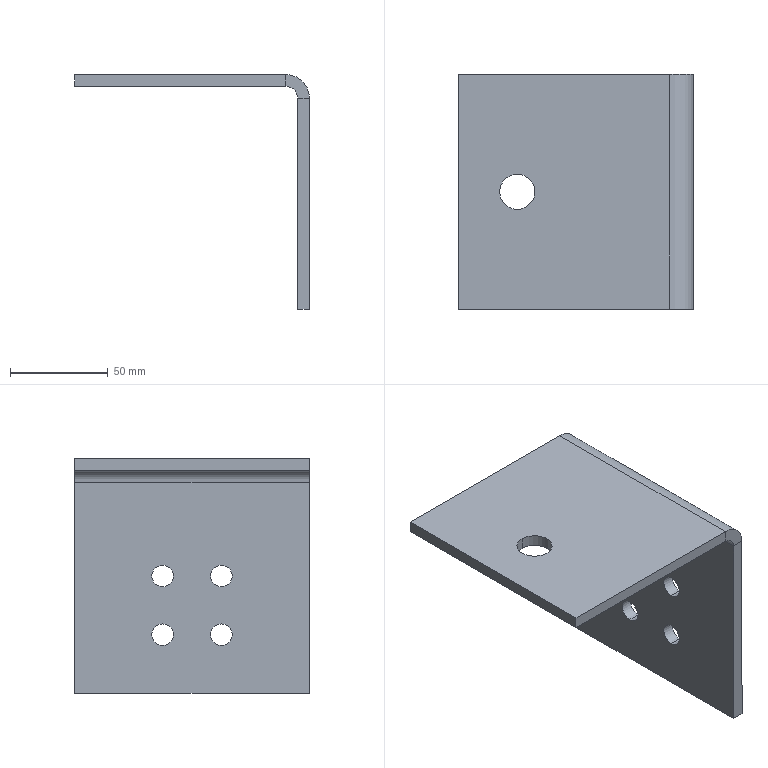Component | SolidWorks | LiftingBentPlate-1 | 1 solid | 24 faces | box 120 x 120 x 120 mm | volume 161891 mm3 | cylinder 12 | plane 12 | commonest cylinder face diameters 11 x8 18 x2 24 x1 12 x1
STEP:
#1=COLOUR_RGB('',0.7922,0.8196,0.9333);
#2=FILL_AREA_STYLE_COLOUR('',#1);
#3=FILL_AREA_STYLE('',(#2));
#4=SURFACE_STYLE_FILL_AREA(#3);
#5=SURFACE_SIDE_STYLE('',(#4));
#6=SURFACE_STYLE_USAGE(.BOTH.,#5);
#7=PRESENTATION_STYLE_ASSIGNMENT((#6));
#8=CARTESIAN_POINT('',(-28.327,8.439,39.587));
#9=VERTEX_POINT('',#8);
#10=CARTESIAN_POINT('',(-28.327,8.439,39.154));
#11=VERTEX_POINT('',#10);
#12=CARTESIAN_POINT('',(-28.327,8.439,39.37));
#13=DIRECTION('',(-1.,0.,0.));
#14=DIRECTION('',(0.,0.,1.));
#15=AXIS2_PLACEMENT_3D('',#12,#13,#14);
#16=CIRCLE('',#15,0.2165);
#17=EDGE_CURVE('',#9,#11,#16,.T.);
#18=ORIENTED_EDGE('',*,*,#17,.T.);
#19=CARTESIAN_POINT('',(-28.091,8.439,39.154));
#20=VERTEX_POINT('',#19);
#21=CARTESIAN_POINT('',(-32.815,8.439,39.154));
#22=DIRECTION('',(1.,-0.,-0.));
#23=VECTOR('',#22,39.37);
#24=LINE('',#21,#23);
#25=EDGE_CURVE('',#11,#20,#24,.T.);
#26=ORIENTED_EDGE('',*,*,#25,.T.);
#27=CARTESIAN_POINT('',(-28.091,8.439,39.587));
#28=VERTEX_POINT('',#27);
#29=CARTESIAN_POINT('',(-28.091,8.439,39.37));
#30=DIRECTION('',(1.,-0.,-0.));
#31=DIRECTION('',(0.,0.,1.));
#32=AXIS2_PLACEMENT_3D('',#29,#30,#31);
#33=CIRCLE('',#32,0.2165);
#34=EDGE_CURVE('',#20,#28,#33,.T.);
#35=ORIENTED_EDGE('',*,*,#34,.T.);
#36=CARTESIAN_POINT('',(-32.815,8.439,39.587));
#37=DIRECTION('',(1.,-0.,-0.));
#38=VECTOR('',#37,39.37);
#39=LINE('',#36,#38);
#40=EDGE_CURVE('',#9,#28,#39,.T.);
#41=ORIENTED_EDGE('',*,*,#40,.F.);
#42=EDGE_LOOP('',(#18,#26,#35,#41));
#43=FACE_OUTER_BOUND('',#42,.T.);
#44=CARTESIAN_POINT('',(-32.815,8.439,39.37));
#45=DIRECTION('',(1.,-0.,-0.));
#46=DIRECTION('',(0.,0.,1.));
#47=AXIS2_PLACEMENT_3D('',#44,#45,#46);
#48=CYLINDRICAL_SURFACE('',#47,0.2165);
#49=ADVANCED_FACE('',(#43),#48,.F.);
#50=CARTESIAN_POINT('',(-28.327,7.258,39.587));
#51=VERTEX_POINT('',#50);
#52=CARTESIAN_POINT('',(-28.327,7.258,39.154));
#53=VERTEX_POINT('',#52);
#54=CARTESIAN_POINT('',(-28.327,7.258,39.37));
#55=DIRECTION('',(-1.,0.,0.));
#56=DIRECTION('',(0.,0.,1.));
#57=AXIS2_PLACEMENT_3D('',#54,#55,#56);
#58=CIRCLE('',#57,0.2165);
#59=EDGE_CURVE('',#51,#53,#58,.T.);
#60=ORIENTED_EDGE('',*,*,#59,.T.);
#61=CARTESIAN_POINT('',(-28.091,7.258,39.154));
#62=VERTEX_POINT('',#61);
#63=CARTESIAN_POINT('',(-32.815,7.258,39.154));
#64=DIRECTION('',(1.,-0.,-0.));
#65=VECTOR('',#64,39.37);
#66=LINE('',#63,#65);
#67=EDGE_CURVE('',#53,#62,#66,.T.);
#68=ORIENTED_EDGE('',*,*,#67,.T.);
#69=CARTESIAN_POINT('',(-28.091,7.258,39.587));
#70=VERTEX_POINT('',#69);
#71=CARTESIAN_POINT('',(-28.091,7.258,39.37));
#72=DIRECTION('',(1.,-0.,-0.));
#73=DIRECTION('',(0.,0.,1.));
#74=AXIS2_PLACEMENT_3D('',#71,#72,#73);
#75=CIRCLE('',#74,0.2165);
#76=EDGE_CURVE('',#62,#70,#75,.T.);
#77=ORIENTED_EDGE('',*,*,#76,.T.);
#78=CARTESIAN_POINT('',(-32.815,7.258,39.587));
#79=DIRECTION('',(1.,-0.,-0.));
#80=VECTOR('',#79,39.37);
#81=LINE('',#78,#80);
#82=EDGE_CURVE('',#51,#70,#81,.T.);
#83=ORIENTED_EDGE('',*,*,#82,.F.);
#84=EDGE_LOOP('',(#60,#68,#77,#83));
#85=FACE_OUTER_BOUND('',#84,.T.);
#86=CARTESIAN_POINT('',(-32.815,7.258,39.37));
#87=DIRECTION('',(1.,-0.,-0.));
#88=DIRECTION('',(0.,0.,1.));
#89=AXIS2_PLACEMENT_3D('',#86,#87,#88);
#90=CYLINDRICAL_SURFACE('',#89,0.2165);
#91=ADVANCED_FACE('',(#85),#90,.F.);
#92=CARTESIAN_POINT('',(-28.327,8.439,40.768));
#93=VERTEX_POINT('',#92);
#94=CARTESIAN_POINT('',(-28.327,8.439,40.335));
#95=VERTEX_POINT('',#94);
#96=CARTESIAN_POINT('',(-28.327,8.439,40.551));
#97=DIRECTION('',(-1.,0.,0.));
#98=DIRECTION('',(0.,0.,1.));
#99=AXIS2_PLACEMENT_3D('',#96,#97,#98);
#100=CIRCLE('',#99,0.2165);
#101=EDGE_CURVE('',#93,#95,#100,.T.);
#102=ORIENTED_EDGE('',*,*,#101,.T.);
#103=CARTESIAN_POINT('',(-28.091,8.439,40.335));
#104=VERTEX_POINT('',#103);
#105=CARTESIAN_POINT('',(-32.815,8.439,40.335));
#106=DIRECTION('',(1.,-0.,-0.));
#107=VECTOR('',#106,39.37);
#108=LINE('',#105,#107);
#109=EDGE_CURVE('',#95,#104,#108,.T.);
#110=ORIENTED_EDGE('',*,*,#109,.T.);
#111=CARTESIAN_POINT('',(-28.091,8.439,40.768));
#112=VERTEX_POINT('',#111);
#113=CARTESIAN_POINT('',(-28.091,8.439,40.551));
#114=DIRECTION('',(1.,-0.,-0.));
#115=DIRECTION('',(0.,0.,1.));
#116=AXIS2_PLACEMENT_3D('',#113,#114,#115);
#117=CIRCLE('',#116,0.2165);
#118=EDGE_CURVE('',#104,#112,#117,.T.);
#119=ORIENTED_EDGE('',*,*,#118,.T.);
#120=CARTESIAN_POINT('',(-32.815,8.439,40.768));
#121=DIRECTION('',(1.,-0.,-0.));
#122=VECTOR('',#121,39.37);
#123=LINE('',#120,#122);
#124=EDGE_CURVE('',#93,#112,#123,.T.);
#125=ORIENTED_EDGE('',*,*,#124,.F.);
#126=EDGE_LOOP('',(#102,#110,#119,#125));
#127=FACE_OUTER_BOUND('',#126,.T.);
#128=CARTESIAN_POINT('',(-32.815,8.439,40.551));
#129=DIRECTION('',(1.,-0.,-0.));
#130=DIRECTION('',(0.,0.,1.));
#131=AXIS2_PLACEMENT_3D('',#128,#129,#130);
#132=CYLINDRICAL_SURFACE('',#131,0.2165);
#133=ADVANCED_FACE('',(#127),#132,.F.);
#134=CARTESIAN_POINT('',(-28.327,7.258,40.768));
#135=VERTEX_POINT('',#134);
#136=CARTESIAN_POINT('',(-28.327,7.258,40.335));
#137=VERTEX_POINT('',#136);
#138=CARTESIAN_POINT('',(-28.327,7.258,40.551));
#139=DIRECTION('',(-1.,0.,0.));
#140=DIRECTION('',(0.,0.,1.));
#141=AXIS2_PLACEMENT_3D('',#138,#139,#140);
#142=CIRCLE('',#141,0.2165);
#143=EDGE_CURVE('',#135,#137,#142,.T.);
#144=ORIENTED_EDGE('',*,*,#143,.T.);
#145=CARTESIAN_POINT('',(-28.091,7.258,40.335));
#146=VERTEX_POINT('',#145);
#147=CARTESIAN_POINT('',(-32.815,7.258,40.335));
#148=DIRECTION('',(1.,-0.,-0.));
#149=VECTOR('',#148,39.37);
#150=LINE('',#147,#149);
#151=EDGE_CURVE('',#137,#146,#150,.T.);
#152=ORIENTED_EDGE('',*,*,#151,.T.);
#153=CARTESIAN_POINT('',(-28.091,7.258,40.768));
#154=VERTEX_POINT('',#153);
#155=CARTESIAN_POINT('',(-28.091,7.258,40.551));
#156=DIRECTION('',(1.,-0.,-0.));
#157=DIRECTION('',(0.,0.,1.));
#158=AXIS2_PLACEMENT_3D('',#155,#156,#157);
#159=CIRCLE('',#158,0.2165);
#160=EDGE_CURVE('',#146,#154,#159,.T.);
#161=ORIENTED_EDGE('',*,*,#160,.T.);
#162=CARTESIAN_POINT('',(-32.815,7.258,40.768));
#163=DIRECTION('',(1.,-0.,-0.));
#164=VECTOR('',#163,39.37);
#165=LINE('',#162,#164);
#166=EDGE_CURVE('',#135,#154,#165,.T.);
#167=ORIENTED_EDGE('',*,*,#166,.F.);
#168=EDGE_LOOP('',(#144,#152,#161,#167));
#169=FACE_OUTER_BOUND('',#168,.T.);
#170=CARTESIAN_POINT('',(-32.815,7.258,40.551));
#171=DIRECTION('',(1.,-0.,-0.));
#172=DIRECTION('',(0.,0.,1.));
#173=AXIS2_PLACEMENT_3D('',#170,#171,#172);
#174=CYLINDRICAL_SURFACE('',#173,0.2165);
#175=ADVANCED_FACE('',(#169),#174,.F.);
#176=CARTESIAN_POINT('',(-31.634,7.494,42.677));
#177=VERTEX_POINT('',#176);
#178=CARTESIAN_POINT('',(-31.634,8.203,42.677));
#179=VERTEX_POINT('',#178);
#180=CARTESIAN_POINT('',(-31.634,7.849,42.677));
#181=DIRECTION('',(-0.,-0.,-1.));
#182=DIRECTION('',(-0.,-1.,0.));
#183=AXIS2_PLACEMENT_3D('',#180,#181,#182);
#184=CIRCLE('',#183,0.3543);
#185=EDGE_CURVE('',#177,#179,#184,.T.);
#186=ORIENTED_EDGE('',*,*,#185,.T.);
#187=CARTESIAN_POINT('',(-31.634,8.203,42.913));
#188=VERTEX_POINT('',#187);
#189=CARTESIAN_POINT('',(-31.634,8.203,38.189));
#190=DIRECTION('',(0.,0.,1.));
#191=VECTOR('',#190,39.37);
#192=LINE('',#189,#191);
#193=EDGE_CURVE('',#179,#188,#192,.T.);
#194=ORIENTED_EDGE('',*,*,#193,.T.);
#195=CARTESIAN_POINT('',(-31.634,7.494,42.913));
#196=VERTEX_POINT('',#195);
#197=CARTESIAN_POINT('',(-31.634,7.849,42.913));
#198=DIRECTION('',(0.,0.,1.));
#199=DIRECTION('',(-0.,-1.,0.));
#200=AXIS2_PLACEMENT_3D('',#197,#198,#199);
#201=CIRCLE('',#200,0.3543);
#202=EDGE_CURVE('',#188,#196,#201,.T.);
#203=ORIENTED_EDGE('',*,*,#202,.T.);
#204=CARTESIAN_POINT('',(-31.634,7.494,38.189));
#205=DIRECTION('',(0.,0.,1.));
#206=VECTOR('',#205,39.37);
#207=LINE('',#204,#206);
#208=EDGE_CURVE('',#177,#196,#207,.T.);
#209=ORIENTED_EDGE('',*,*,#208,.F.);
#210=EDGE_LOOP('',(#186,#194,#203,#209));
#211=FACE_OUTER_BOUND('',#210,.T.);
#212=CARTESIAN_POINT('',(-31.634,7.849,38.189));
#213=DIRECTION('',(0.,0.,1.));
#214=DIRECTION('',(-0.,-1.,0.));
#215=AXIS2_PLACEMENT_3D('',#212,#213,#214);
#216=CYLINDRICAL_SURFACE('',#215,0.3543);
#217=ADVANCED_FACE('',(#211),#216,.F.);
#218=CARTESIAN_POINT('',(-28.091,5.486,42.441));
#219=VERTEX_POINT('',#218);
#220=CARTESIAN_POINT('',(-28.327,5.486,42.441));
#221=VERTEX_POINT('',#220);
#222=CARTESIAN_POINT('',(-28.091,5.486,42.441));
#223=DIRECTION('',(-1.,0.,0.));
#224=VECTOR('',#223,39.37);
#225=LINE('',#222,#224);
#226=EDGE_CURVE('',#219,#221,#225,.T.);
#227=ORIENTED_EDGE('',*,*,#226,.F.);
#228=CARTESIAN_POINT('',(-28.563,5.486,42.913));
#229=VERTEX_POINT('',#228);
#230=CARTESIAN_POINT('',(-28.563,5.486,42.441));
#231=DIRECTION('',(0.,1.,-0.));
#232=DIRECTION('',(1.,-0.,0.));
#233=AXIS2_PLACEMENT_3D('',#230,#231,#232);
#234=CIRCLE('',#233,0.4724);
#235=EDGE_CURVE('',#229,#219,#234,.T.);
#236=ORIENTED_EDGE('',*,*,#235,.F.);
#237=CARTESIAN_POINT('',(-28.563,5.486,42.677));
#238=VERTEX_POINT('',#237);
#239=CARTESIAN_POINT('',(-28.563,5.486,42.677));
#240=DIRECTION('',(0.,0.,1.));
#241=VECTOR('',#240,39.37);
#242=LINE('',#239,#241);
#243=EDGE_CURVE('',#238,#229,#242,.T.);
#244=ORIENTED_EDGE('',*,*,#243,.F.);
#245=CARTESIAN_POINT('',(-28.563,5.486,42.441));
#246=DIRECTION('',(0.,1.,-0.));
#247=DIRECTION('',(1.,-0.,0.));
#248=AXIS2_PLACEMENT_3D('',#245,#246,#247);
#249=CIRCLE('',#248,0.2362);
#250=EDGE_CURVE('',#238,#221,#249,.T.);
#251=ORIENTED_EDGE('',*,*,#250,.T.);
#252=EDGE_LOOP('',(#227,#236,#244,#251));
#253=FACE_OUTER_BOUND('',#252,.T.);
#254=CARTESIAN_POINT('',(-28.091,5.486,42.441));
#255=DIRECTION('',(-0.,-1.,0.));
#256=DIRECTION('',(1.,-0.,-0.));
#257=AXIS2_PLACEMENT_3D('',#254,#255,#256);
#258=PLANE('',#257);
#259=ADVANCED_FACE('',(#253),#258,.T.);
#260=CARTESIAN_POINT('',(-28.091,5.486,38.189));
#261=VERTEX_POINT('',#260);
#262=CARTESIAN_POINT('',(-28.091,5.486,42.913));
#263=DIRECTION('',(-0.,-0.,-1.));
#264=VECTOR('',#263,39.37);
#265=LINE('',#262,#264);
#266=EDGE_CURVE('',#219,#261,#265,.T.);
#267=ORIENTED_EDGE('',*,*,#266,.F.);
#268=ORIENTED_EDGE('',*,*,#226,.T.);
#269=CARTESIAN_POINT('',(-28.327,5.486,38.189));
#270=VERTEX_POINT('',#269);
#271=CARTESIAN_POINT('',(-28.327,5.486,42.913));
#272=DIRECTION('',(-0.,-0.,-1.));
#273=VECTOR('',#272,39.37);
#274=LINE('',#271,#273);
#275=EDGE_CURVE('',#221,#270,#274,.T.);
#276=ORIENTED_EDGE('',*,*,#275,.T.);
#277=CARTESIAN_POINT('',(-28.091,5.486,38.189));
#278=DIRECTION('',(-1.,0.,0.));
#279=VECTOR('',#278,39.37);
#280=LINE('',#277,#279);
#281=EDGE_CURVE('',#261,#270,#280,.T.);
#282=ORIENTED_EDGE('',*,*,#281,.F.);
#283=EDGE_LOOP('',(#267,#268,#276,#282));
#284=FACE_OUTER_BOUND('',#283,.T.);
#285=CARTESIAN_POINT('',(-28.563,5.486,42.677));
#286=DIRECTION('',(-0.,-1.,0.));
#287=DIRECTION('',(1.,-0.,-0.));
#288=AXIS2_PLACEMENT_3D('',#285,#286,#287);
#289=PLANE('',#288);
#290=ADVANCED_FACE('',(#284),#289,.T.);
#291=CARTESIAN_POINT('',(-28.563,10.211,42.913));
#292=VERTEX_POINT('',#291);
#293=CARTESIAN_POINT('',(-28.563,10.211,42.677));
#294=VERTEX_POINT('',#293);
#295=CARTESIAN_POINT('',(-28.563,10.211,42.913));
#296=DIRECTION('',(-0.,-0.,-1.));
#297=VECTOR('',#296,39.37);
#298=LINE('',#295,#297);
#299=EDGE_CURVE('',#292,#294,#298,.T.);
#300=ORIENTED_EDGE('',*,*,#299,.F.);
#301=CARTESIAN_POINT('',(-28.091,10.211,42.441));
#302=VERTEX_POINT('',#301);
#303=CARTESIAN_POINT('',(-28.563,10.211,42.441));
#304=DIRECTION('',(0.,1.,-0.));
#305=DIRECTION('',(1.,-0.,0.));
#306=AXIS2_PLACEMENT_3D('',#303,#304,#305);
#307=CIRCLE('',#306,0.4724);
#308=EDGE_CURVE('',#292,#302,#307,.T.);
#309=ORIENTED_EDGE('',*,*,#308,.T.);
#310=CARTESIAN_POINT('',(-28.327,10.211,42.441));
#311=VERTEX_POINT('',#310);
#312=CARTESIAN_POINT('',(-28.327,10.211,42.441));
#313=DIRECTION('',(1.,-0.,-0.));
#314=VECTOR('',#313,39.37);
#315=LINE('',#312,#314);
#316=EDGE_CURVE('',#311,#302,#315,.T.);
#317=ORIENTED_EDGE('',*,*,#316,.F.);
#318=CARTESIAN_POINT('',(-28.563,10.211,42.441));
#319=DIRECTION('',(0.,1.,-0.));
#320=DIRECTION('',(1.,-0.,0.));
#321=AXIS2_PLACEMENT_3D('',#318,#319,#320);
#322=CIRCLE('',#321,0.2362);
#323=EDGE_CURVE('',#294,#311,#322,.T.);
#324=ORIENTED_EDGE('',*,*,#323,.F.);
#325=EDGE_LOOP('',(#300,#309,#317,#324));
#326=FACE_OUTER_BOUND('',#325,.T.);
#327=CARTESIAN_POINT('',(-28.563,10.211,42.913));
#328=DIRECTION('',(0.,1.,-0.));
#329=DIRECTION('',(-1.,0.,0.));
#330=AXIS2_PLACEMENT_3D('',#327,#328,#329);
#331=PLANE('',#330);
#332=ADVANCED_FACE('',(#326),#331,.T.);
#333=CARTESIAN_POINT('',(-32.815,10.211,42.913));
#334=VERTEX_POINT('',#333);
#335=CARTESIAN_POINT('',(-32.815,10.211,42.913));
#336=DIRECTION('',(1.,-0.,-0.));
#337=VECTOR('',#336,39.37);
#338=LINE('',#335,#337);
#339=EDGE_CURVE('',#334,#292,#338,.T.);
#340=ORIENTED_EDGE('',*,*,#339,.T.);
#341=ORIENTED_EDGE('',*,*,#299,.T.);
#342=CARTESIAN_POINT('',(-32.815,10.211,42.677));
#343=VERTEX_POINT('',#342);
#344=CARTESIAN_POINT('',(-32.815,10.211,42.677));
#345=DIRECTION('',(1.,-0.,-0.));
#346=VECTOR('',#345,39.37);
#347=LINE('',#344,#346);
#348=EDGE_CURVE('',#343,#294,#347,.T.);
#349=ORIENTED_EDGE('',*,*,#348,.F.);
#350=CARTESIAN_POINT('',(-32.815,10.211,42.677));
#351=DIRECTION('',(0.,0.,1.));
#352=VECTOR('',#351,39.37);
#353=LINE('',#350,#352);
#354=EDGE_CURVE('',#343,#334,#353,.T.);
#355=ORIENTED_EDGE('',*,*,#354,.T.);
#356=EDGE_LOOP('',(#340,#341,#349,#355));
#357=FACE_OUTER_BOUND('',#356,.T.);
#358=CARTESIAN_POINT('',(-28.327,10.211,42.441));
#359=DIRECTION('',(0.,1.,-0.));
#360=DIRECTION('',(-1.,0.,0.));
#361=AXIS2_PLACEMENT_3D('',#358,#359,#360);
#362=PLANE('',#361);
#363=ADVANCED_FACE('',(#357),#362,.T.);
#364=ORIENTED_EDGE('',*,*,#17,.F.);
#365=CARTESIAN_POINT('',(-28.327,8.439,39.37));
#366=DIRECTION('',(-1.,0.,0.));
#367=DIRECTION('',(0.,0.,1.));
#368=AXIS2_PLACEMENT_3D('',#365,#366,#367);
#369=CIRCLE('',#368,0.2165);
#370=EDGE_CURVE('',#11,#9,#369,.T.);
#371=ORIENTED_EDGE('',*,*,#370,.F.);
#372=EDGE_LOOP('',(#364,#371));
#373=FACE_BOUND('',#372,.T.);
#374=ORIENTED_EDGE('',*,*,#59,.F.);
#375=CARTESIAN_POINT('',(-28.327,7.258,39.37));
#376=DIRECTION('',(-1.,0.,0.));
#377=DIRECTION('',(0.,0.,1.));
#378=AXIS2_PLACEMENT_3D('',#375,#376,#377);
#379=CIRCLE('',#378,0.2165);
#380=EDGE_CURVE('',#53,#51,#379,.T.);
#381=ORIENTED_EDGE('',*,*,#380,.F.);
#382=EDGE_LOOP('',(#374,#381));
#383=FACE_BOUND('',#382,.T.);
#384=ORIENTED_EDGE('',*,*,#101,.F.);
#385=CARTESIAN_POINT('',(-28.327,8.439,40.551));
#386=DIRECTION('',(-1.,0.,0.));
#387=DIRECTION('',(0.,0.,1.));
#388=AXIS2_PLACEMENT_3D('',#385,#386,#387);
#389=CIRCLE('',#388,0.2165);
#390=EDGE_CURVE('',#95,#93,#389,.T.);
#391=ORIENTED_EDGE('',*,*,#390,.F.);
#392=EDGE_LOOP('',(#384,#391));
#393=FACE_BOUND('',#392,.T.);
#394=ORIENTED_EDGE('',*,*,#143,.F.);
#395=CARTESIAN_POINT('',(-28.327,7.258,40.551));
#396=DIRECTION('',(-1.,0.,0.));
#397=DIRECTION('',(0.,0.,1.));
#398=AXIS2_PLACEMENT_3D('',#395,#396,#397);
#399=CIRCLE('',#398,0.2165);
#400=EDGE_CURVE('',#137,#135,#399,.T.);
#401=ORIENTED_EDGE('',*,*,#400,.F.);
#402=EDGE_LOOP('',(#394,#401));
#403=FACE_BOUND('',#402,.T.);
#404=CARTESIAN_POINT('',(-28.327,10.211,38.189));
#405=VERTEX_POINT('',#404);
#406=CARTESIAN_POINT('',(-28.327,10.211,42.913));
#407=DIRECTION('',(-0.,-0.,-1.));
#408=VECTOR('',#407,39.37);
#409=LINE('',#406,#408);
#410=EDGE_CURVE('',#311,#405,#409,.T.);
#411=ORIENTED_EDGE('',*,*,#410,.T.);
#412=CARTESIAN_POINT('',(-28.327,5.486,38.189));
#413=DIRECTION('',(0.,1.,-0.));
#414=VECTOR('',#413,39.37);
#415=LINE('',#412,#414);
#416=EDGE_CURVE('',#270,#405,#415,.T.);
#417=ORIENTED_EDGE('',*,*,#416,.F.);
#418=ORIENTED_EDGE('',*,*,#275,.F.);
#419=CARTESIAN_POINT('',(-28.327,5.486,42.441));
#420=DIRECTION('',(0.,1.,-0.));
#421=VECTOR('',#420,39.37);
#422=LINE('',#419,#421);
#423=EDGE_CURVE('',#221,#311,#422,.T.);
#424=ORIENTED_EDGE('',*,*,#423,.T.);
#425=EDGE_LOOP('',(#411,#417,#418,#424));
#426=FACE_OUTER_BOUND('',#425,.T.);
#427=CARTESIAN_POINT('',(-28.327,5.486,42.913));
#428=DIRECTION('',(1.,-0.,-0.));
#429=DIRECTION('',(0.,0.,1.));
#430=AXIS2_PLACEMENT_3D('',#427,#428,#429);
#431=PLANE('',#430);
#432=ADVANCED_FACE('',(#373,#383,#393,#403,#426),#431,.F.);
#433=CARTESIAN_POINT('',(-28.091,10.211,38.189));
#434=VERTEX_POINT('',#433);
#435=CARTESIAN_POINT('',(-28.091,10.211,38.189));
#436=DIRECTION('',(-1.,0.,0.));
#437=VECTOR('',#436,39.37);
#438=LINE('',#435,#437);
#439=EDGE_CURVE('',#434,#405,#438,.T.);
#440=ORIENTED_EDGE('',*,*,#439,.F.);
#441=CARTESIAN_POINT('',(-28.091,5.486,38.189));
#442=DIRECTION('',(0.,1.,-0.));
#443=VECTOR('',#442,39.37);
#444=LINE('',#441,#443);
#445=EDGE_CURVE('',#261,#434,#444,.T.);
#446=ORIENTED_EDGE('',*,*,#445,.F.);
#447=ORIENTED_EDGE('',*,*,#281,.T.);
#448=ORIENTED_EDGE('',*,*,#416,.T.);
#449=EDGE_LOOP('',(#440,#446,#447,#448));
#450=FACE_OUTER_BOUND('',#449,.T.);
#451=CARTESIAN_POINT('',(-28.091,5.486,38.189));
#452=DIRECTION('',(-0.,-0.,-1.));
#453=DIRECTION('',(0.,1.,-0.));
#454=AXIS2_PLACEMENT_3D('',#451,#452,#453);
#455=PLANE('',#454);
#456=ADVANCED_FACE('',(#450),#455,.T.);
#457=CARTESIAN_POINT('',(-28.091,8.439,39.37));
#458=DIRECTION('',(1.,-0.,-0.));
#459=DIRECTION('',(0.,0.,1.));
#460=AXIS2_PLACEMENT_3D('',#457,#458,#459);
#461=CIRCLE('',#460,0.2165);
#462=EDGE_CURVE('',#28,#20,#461,.T.);
#463=ORIENTED_EDGE('',*,*,#462,.F.);
#464=ORIENTED_EDGE('',*,*,#34,.F.);
#465=EDGE_LOOP('',(#463,#464));
#466=FACE_BOUND('',#465,.T.);
#467=CARTESIAN_POINT('',(-28.091,7.258,39.37));
#468=DIRECTION('',(1.,-0.,-0.));
#469=DIRECTION('',(0.,0.,1.));
#470=AXIS2_PLACEMENT_3D('',#467,#468,#469);
#471=CIRCLE('',#470,0.2165);
#472=EDGE_CURVE('',#70,#62,#471,.T.);
#473=ORIENTED_EDGE('',*,*,#472,.F.);
#474=ORIENTED_EDGE('',*,*,#76,.F.);
#475=EDGE_LOOP('',(#473,#474));
#476=FACE_BOUND('',#475,.T.);
#477=CARTESIAN_POINT('',(-28.091,8.439,40.551));
#478=DIRECTION('',(1.,-0.,-0.));
#479=DIRECTION('',(0.,0.,1.));
#480=AXIS2_PLACEMENT_3D('',#477,#478,#479);
#481=CIRCLE('',#480,0.2165);
#482=EDGE_CURVE('',#112,#104,#481,.T.);
#483=ORIENTED_EDGE('',*,*,#482,.F.);
#484=ORIENTED_EDGE('',*,*,#118,.F.);
#485=EDGE_LOOP('',(#483,#484));
#486=FACE_BOUND('',#485,.T.);
#487=CARTESIAN_POINT('',(-28.091,7.258,40.551));
#488=DIRECTION('',(1.,-0.,-0.));
#489=DIRECTION('',(0.,0.,1.));
#490=AXIS2_PLACEMENT_3D('',#487,#488,#489);
#491=CIRCLE('',#490,0.2165);
#492=EDGE_CURVE('',#154,#146,#491,.T.);
#493=ORIENTED_EDGE('',*,*,#492,.F.);
#494=ORIENTED_EDGE('',*,*,#160,.F.);
#495=EDGE_LOOP('',(#493,#494));
#496=FACE_BOUND('',#495,.T.);
#497=CARTESIAN_POINT('',(-28.091,10.211,42.913));
#498=DIRECTION('',(-0.,-0.,-1.));
#499=VECTOR('',#498,39.37);
#500=LINE('',#497,#499);
#501=EDGE_CURVE('',#302,#434,#500,.T.);
#502=ORIENTED_EDGE('',*,*,#501,.F.);
#503=CARTESIAN_POINT('',(-28.091,5.486,42.441));
#504=DIRECTION('',(0.,1.,-0.));
#505=VECTOR('',#504,39.37);
#506=LINE('',#503,#505);
#507=EDGE_CURVE('',#219,#302,#506,.T.);
#508=ORIENTED_EDGE('',*,*,#507,.F.);
#509=ORIENTED_EDGE('',*,*,#266,.T.);
#510=ORIENTED_EDGE('',*,*,#445,.T.);
#511=EDGE_LOOP('',(#502,#508,#509,#510));
#512=FACE_OUTER_BOUND('',#511,.T.);
#513=CARTESIAN_POINT('',(-28.091,5.486,42.913));
#514=DIRECTION('',(1.,-0.,-0.));
#515=DIRECTION('',(0.,0.,1.));
#516=AXIS2_PLACEMENT_3D('',#513,#514,#515);
#517=PLANE('',#516);
#518=ADVANCED_FACE('',(#466,#476,#486,#496,#512),#517,.T.);
#519=ORIENTED_EDGE('',*,*,#308,.F.);
#520=CARTESIAN_POINT('',(-28.563,5.486,42.913));
#521=DIRECTION('',(0.,1.,-0.));
#522=VECTOR('',#521,39.37);
#523=LINE('',#520,#522);
#524=EDGE_CURVE('',#229,#292,#523,.T.);
#525=ORIENTED_EDGE('',*,*,#524,.F.);
#526=ORIENTED_EDGE('',*,*,#235,.T.);
#527=ORIENTED_EDGE('',*,*,#507,.T.);
#528=EDGE_LOOP('',(#519,#525,#526,#527));
#529=FACE_OUTER_BOUND('',#528,.T.);
#530=CARTESIAN_POINT('',(-28.563,5.486,42.441));
#531=DIRECTION('',(0.,1.,-0.));
#532=DIRECTION('',(-1.,0.,0.));
#533=AXIS2_PLACEMENT_3D('',#530,#531,#532);
#534=CYLINDRICAL_SURFACE('',#533,0.4724);
#535=ADVANCED_FACE('',(#529),#534,.T.);
#536=CARTESIAN_POINT('',(-31.634,7.849,42.913));
#537=DIRECTION('',(0.,0.,1.));
#538=DIRECTION('',(-0.,-1.,0.));
#539=AXIS2_PLACEMENT_3D('',#536,#537,#538);
#540=CIRCLE('',#539,0.3543);
#541=EDGE_CURVE('',#196,#188,#540,.T.);
#542=ORIENTED_EDGE('',*,*,#541,.F.);
#543=ORIENTED_EDGE('',*,*,#202,.F.);
#544=EDGE_LOOP('',(#542,#543));
#545=FACE_BOUND('',#544,.T.);
#546=ORIENTED_EDGE('',*,*,#339,.F.);
#547=CARTESIAN_POINT('',(-32.815,5.486,42.913));
#548=VERTEX_POINT('',#547);
#549=CARTESIAN_POINT('',(-32.815,5.486,42.913));
#550=DIRECTION('',(0.,1.,-0.));
#551=VECTOR('',#550,39.37);
#552=LINE('',#549,#551);
#553=EDGE_CURVE('',#548,#334,#552,.T.);
#554=ORIENTED_EDGE('',*,*,#553,.F.);
#555=CARTESIAN_POINT('',(-32.815,5.486,42.913));
#556=DIRECTION('',(1.,-0.,-0.));
#557=VECTOR('',#556,39.37);
#558=LINE('',#555,#557);
#559=EDGE_CURVE('',#548,#229,#558,.T.);
#560=ORIENTED_EDGE('',*,*,#559,.T.);
#561=ORIENTED_EDGE('',*,*,#524,.T.);
#562=EDGE_LOOP('',(#546,#554,#560,#561));
#563=FACE_OUTER_BOUND('',#562,.T.);
#564=CARTESIAN_POINT('',(-32.815,5.486,42.913));
#565=DIRECTION('',(0.,0.,1.));
#566=DIRECTION('',(-0.,-1.,0.));
#567=AXIS2_PLACEMENT_3D('',#564,#565,#566);
#568=PLANE('',#567);
#569=ADVANCED_FACE('',(#545,#563),#568,.T.);
#570=ORIENTED_EDGE('',*,*,#354,.F.);
#571=CARTESIAN_POINT('',(-32.815,5.486,42.677));
#572=VERTEX_POINT('',#571);
#573=CARTESIAN_POINT('',(-32.815,5.486,42.677));
#574=DIRECTION('',(0.,1.,-0.));
#575=VECTOR('',#574,39.37);
#576=LINE('',#573,#575);
#577=EDGE_CURVE('',#572,#343,#576,.T.);
#578=ORIENTED_EDGE('',*,*,#577,.F.);
#579=CARTESIAN_POINT('',(-32.815,5.486,42.677));
#580=DIRECTION('',(0.,0.,1.));
#581=VECTOR('',#580,39.37);
#582=LINE('',#579,#581);
#583=EDGE_CURVE('',#572,#548,#582,.T.);
#584=ORIENTED_EDGE('',*,*,#583,.T.);
#585=ORIENTED_EDGE('',*,*,#553,.T.);
#586=EDGE_LOOP('',(#570,#578,#584,#585));
#587=FACE_OUTER_BOUND('',#586,.T.);
#588=CARTESIAN_POINT('',(-32.815,5.486,42.677));
#589=DIRECTION('',(-1.,0.,0.));
#590=DIRECTION('',(-0.,-1.,0.));
#591=AXIS2_PLACEMENT_3D('',#588,#589,#590);
#592=PLANE('',#591);
#593=ADVANCED_FACE('',(#587),#592,.T.);
#594=ORIENTED_EDGE('',*,*,#185,.F.);
#595=CARTESIAN_POINT('',(-31.634,7.849,42.677));
#596=DIRECTION('',(-0.,-0.,-1.));
#597=DIRECTION('',(0.,-1.,0.));
#598=AXIS2_PLACEMENT_3D('',#595,#596,#597);
#599=CIRCLE('',#598,0.3543);
#600=EDGE_CURVE('',#179,#177,#599,.T.);
#601=ORIENTED_EDGE('',*,*,#600,.F.);
#602=EDGE_LOOP('',(#594,#601));
#603=FACE_BOUND('',#602,.T.);
#604=ORIENTED_EDGE('',*,*,#348,.T.);
#605=CARTESIAN_POINT('',(-28.563,5.486,42.677));
#606=DIRECTION('',(0.,1.,-0.));
#607=VECTOR('',#606,39.37);
#608=LINE('',#605,#607);
#609=EDGE_CURVE('',#238,#294,#608,.T.);
#610=ORIENTED_EDGE('',*,*,#609,.F.);
#611=CARTESIAN_POINT('',(-32.815,5.486,42.677));
#612=DIRECTION('',(1.,-0.,-0.));
#613=VECTOR('',#612,39.37);
#614=LINE('',#611,#613);
#615=EDGE_CURVE('',#572,#238,#614,.T.);
#616=ORIENTED_EDGE('',*,*,#615,.F.);
#617=ORIENTED_EDGE('',*,*,#577,.T.);
#618=EDGE_LOOP('',(#604,#610,#616,#617));
#619=FACE_OUTER_BOUND('',#618,.T.);
#620=CARTESIAN_POINT('',(-32.815,5.486,42.677));
#621=DIRECTION('',(0.,0.,1.));
#622=DIRECTION('',(-0.,-1.,0.));
#623=AXIS2_PLACEMENT_3D('',#620,#621,#622);
#624=PLANE('',#623);
#625=ADVANCED_FACE('',(#603,#619),#624,.F.);
#626=ORIENTED_EDGE('',*,*,#323,.T.);
#627=ORIENTED_EDGE('',*,*,#423,.F.);
#628=ORIENTED_EDGE('',*,*,#250,.F.);
#629=ORIENTED_EDGE('',*,*,#609,.T.);
#630=EDGE_LOOP('',(#626,#627,#628,#629));
#631=FACE_OUTER_BOUND('',#630,.T.);
#632=CARTESIAN_POINT('',(-28.563,5.486,42.441));
#633=DIRECTION('',(0.,1.,-0.));
#634=DIRECTION('',(-1.,0.,0.));
#635=AXIS2_PLACEMENT_3D('',#632,#633,#634);
#636=CYLINDRICAL_SURFACE('',#635,0.2362);
#637=ADVANCED_FACE('',(#631),#636,.F.);
#638=ORIENTED_EDGE('',*,*,#615,.T.);
#639=ORIENTED_EDGE('',*,*,#243,.T.);
#640=ORIENTED_EDGE('',*,*,#559,.F.);
#641=ORIENTED_EDGE('',*,*,#583,.F.);
#642=EDGE_LOOP('',(#638,#639,#640,#641));
#643=FACE_OUTER_BOUND('',#642,.T.);
#644=CARTESIAN_POINT('',(-28.563,5.486,42.441));
#645=DIRECTION('',(-0.,-1.,0.));
#646=DIRECTION('',(1.,-0.,-0.));
#647=AXIS2_PLACEMENT_3D('',#644,#645,#646);
#648=PLANE('',#647);
#649=ADVANCED_FACE('',(#643),#648,.T.);
#650=ORIENTED_EDGE('',*,*,#410,.F.);
#651=ORIENTED_EDGE('',*,*,#316,.T.);
#652=ORIENTED_EDGE('',*,*,#501,.T.);
#653=ORIENTED_EDGE('',*,*,#439,.T.);
#654=EDGE_LOOP('',(#650,#651,#652,#653));
#655=FACE_OUTER_BOUND('',#654,.T.);
#656=CARTESIAN_POINT('',(-28.563,10.211,42.441));
#657=DIRECTION('',(-0.,-1.,0.));
#658=DIRECTION('',(1.,-0.,-0.));
#659=AXIS2_PLACEMENT_3D('',#656,#657,#658);
#660=PLANE('',#659);
#661=ADVANCED_FACE('',(#655),#660,.F.);
#662=ORIENTED_EDGE('',*,*,#193,.F.);
#663=ORIENTED_EDGE('',*,*,#600,.T.);
#664=ORIENTED_EDGE('',*,*,#208,.T.);
#665=ORIENTED_EDGE('',*,*,#541,.T.);
#666=EDGE_LOOP('',(#662,#663,#664,#665));
#667=FACE_OUTER_BOUND('',#666,.T.);
#668=CARTESIAN_POINT('',(-31.634,7.849,38.189));
#669=DIRECTION('',(0.,0.,1.));
#670=DIRECTION('',(-0.,-1.,0.));
#671=AXIS2_PLACEMENT_3D('',#668,#669,#670);
#672=CYLINDRICAL_SURFACE('',#671,0.3543);
#673=ADVANCED_FACE('',(#667),#672,.F.);
#674=ORIENTED_EDGE('',*,*,#151,.F.);
#675=ORIENTED_EDGE('',*,*,#400,.T.);
#676=ORIENTED_EDGE('',*,*,#166,.T.);
#677=ORIENTED_EDGE('',*,*,#492,.T.);
#678=EDGE_LOOP('',(#674,#675,#676,#677));
#679=FACE_OUTER_BOUND('',#678,.T.);
#680=CARTESIAN_POINT('',(-32.815,7.258,40.551));
#681=DIRECTION('',(1.,-0.,-0.));
#682=DIRECTION('',(0.,0.,1.));
#683=AXIS2_PLACEMENT_3D('',#680,#681,#682);
#684=CYLINDRICAL_SURFACE('',#683,0.2165);
#685=ADVANCED_FACE('',(#679),#684,.F.);
#686=ORIENTED_EDGE('',*,*,#109,.F.);
#687=ORIENTED_EDGE('',*,*,#390,.T.);
#688=ORIENTED_EDGE('',*,*,#124,.T.);
#689=ORIENTED_EDGE('',*,*,#482,.T.);
#690=EDGE_LOOP('',(#686,#687,#688,#689));
#691=FACE_OUTER_BOUND('',#690,.T.);
#692=CARTESIAN_POINT('',(-32.815,8.439,40.551));
#693=DIRECTION('',(1.,-0.,-0.));
#694=DIRECTION('',(0.,0.,1.));
#695=AXIS2_PLACEMENT_3D('',#692,#693,#694);
#696=CYLINDRICAL_SURFACE('',#695,0.2165);
#697=ADVANCED_FACE('',(#691),#696,.F.);
#698=ORIENTED_EDGE('',*,*,#67,.F.);
#699=ORIENTED_EDGE('',*,*,#380,.T.);
#700=ORIENTED_EDGE('',*,*,#82,.T.);
#701=ORIENTED_EDGE('',*,*,#472,.T.);
#702=EDGE_LOOP('',(#698,#699,#700,#701));
#703=FACE_OUTER_BOUND('',#702,.T.);
#704=CARTESIAN_POINT('',(-32.815,7.258,39.37));
#705=DIRECTION('',(1.,-0.,-0.));
#706=DIRECTION('',(0.,0.,1.));
#707=AXIS2_PLACEMENT_3D('',#704,#705,#706);
#708=CYLINDRICAL_SURFACE('',#707,0.2165);
#709=ADVANCED_FACE('',(#703),#708,.F.);
#710=ORIENTED_EDGE('',*,*,#25,.F.);
#711=ORIENTED_EDGE('',*,*,#370,.T.);
#712=ORIENTED_EDGE('',*,*,#40,.T.);
#713=ORIENTED_EDGE('',*,*,#462,.T.);
#714=EDGE_LOOP('',(#710,#711,#712,#713));
#715=FACE_OUTER_BOUND('',#714,.T.);
#716=CARTESIAN_POINT('',(-32.815,8.439,39.37));
#717=DIRECTION('',(1.,-0.,-0.));
#718=DIRECTION('',(0.,0.,1.));
#719=AXIS2_PLACEMENT_3D('',#716,#717,#718);
#720=CYLINDRICAL_SURFACE('',#719,0.2165);
#721=ADVANCED_FACE('',(#715),#720,.F.);
#722=CLOSED_SHELL('',(#49,#91,#133,#175,#217,#259,#290,#332,#363,#432,#456,#518,#535,#569,#593,#625,#637,#649,#661,#673,#685,#697,#709,#721));
#723=MANIFOLD_SOLID_BREP('',#722);
#724=STYLED_ITEM('',(#7),#723);
#725=(LENGTH_UNIT()NAMED_UNIT(*)SI_UNIT($,.METRE.));
#726=LENGTH_MEASURE_WITH_UNIT(LENGTH_MEASURE(0.0254),#725);
#727=DIMENSIONAL_EXPONENTS(1.,0.,0.,0.,0.,0.,0.);
#728=(CONVERSION_BASED_UNIT('',#726)LENGTH_UNIT()NAMED_UNIT(#727));
#729=UNCERTAINTY_MEASURE_WITH_UNIT(LENGTH_MEASURE(0.00001),#728,'','');
#730=(NAMED_UNIT(*)PLANE_ANGLE_UNIT()SI_UNIT($,.RADIAN.));
#731=(NAMED_UNIT(*)SI_UNIT($,.STERADIAN.)SOLID_ANGLE_UNIT());
#732=(GEOMETRIC_REPRESENTATION_CONTEXT(3)GLOBAL_UNCERTAINTY_ASSIGNED_CONTEXT((#729))GLOBAL_UNIT_ASSIGNED_CONTEXT((#728,#730,#731))REPRESENTATION_CONTEXT('',''));
#733=MECHANICAL_DESIGN_GEOMETRIC_PRESENTATION_REPRESENTATION('',(#724),#732);
#734=PRESENTATION_LAYER_ASSIGNMENT('','',(#724));
#735=CARTESIAN_POINT('',(0.,0.,0.));
#736=DIRECTION('',(0.,0.,1.));
#737=DIRECTION('',(1.,0.,0.));
#738=AXIS2_PLACEMENT_3D('',#735,#736,#737);
#739=(LENGTH_UNIT()NAMED_UNIT(*)SI_UNIT($,.METRE.));
#740=LENGTH_MEASURE_WITH_UNIT(LENGTH_MEASURE(0.0254),#739);
#741=DIMENSIONAL_EXPONENTS(1.,0.,0.,0.,0.,0.,0.);
#742=(CONVERSION_BASED_UNIT('',#740)LENGTH_UNIT()NAMED_UNIT(#741));
#743=UNCERTAINTY_MEASURE_WITH_UNIT(LENGTH_MEASURE(0.00001),#742,'','');
#744=(NAMED_UNIT(*)PLANE_ANGLE_UNIT()SI_UNIT($,.RADIAN.));
#745=(NAMED_UNIT(*)SI_UNIT($,.STERADIAN.)SOLID_ANGLE_UNIT());
#746=(GEOMETRIC_REPRESENTATION_CONTEXT(3)GLOBAL_UNCERTAINTY_ASSIGNED_CONTEXT((#743))GLOBAL_UNIT_ASSIGNED_CONTEXT((#742,#744,#745))REPRESENTATION_CONTEXT('',''));
#747=ADVANCED_BREP_SHAPE_REPRESENTATION('',(#723,#738),#746);